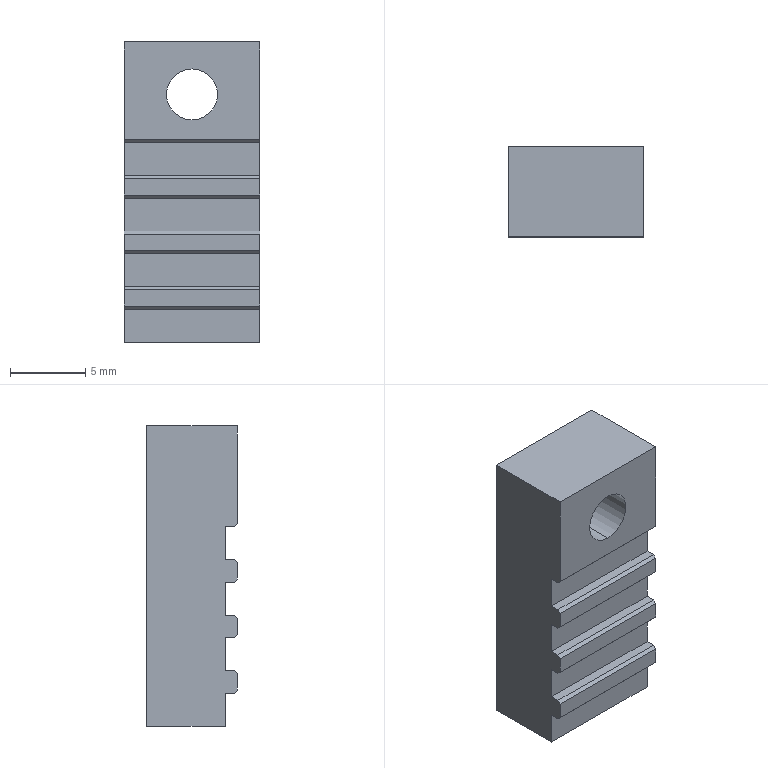Part | SolidWorks | mm | material A6061 | 1 solid | 32 faces | box 9 x 6 x 20 mm | volume 896 mm3 | plane 28 | cylinder 4 | commonest cylinder face diameters 6 x2 3.4 x2
Drawing notes:
0.20 X 45° CHAMFER TYP 7 PLCS - ALL GROOVE EDGES | from the solid: 7 inclined planes at 45° to y/z, size 9.0 x 0.2 x 0.2, at z=2.2, 3.5, 5.9, 7.2, 9.6, 10.9, 13.3
build123d program:
from build123d import *

# Parameters (mm, degrees)
SKETCH1_W                                       = 9
SKETCH1_H                                       = 20
BOSS_EXTRUDE1_DEPTH                             = 6
M3_HEX_SOCKET_HEAD_CAP_SCREW_CBORE1_D           = 3.4
M3_HEX_SOCKET_HEAD_CAP_SCREW_CBORE1_CBORE_D     = 6
M3_HEX_SOCKET_HEAD_CAP_SCREW_CBORE1_CBORE_DEPTH = 3.4
SKETCH5_W                                       = 2.2
SKETCH5_H                                       = 1.6
CUT_EXTRUDE1_DEPTH                              = 10
LPATTERN1_COUNT                                 = 4
LPATTERN1_PITCH                                 = 3.7
CHAMFER1_SIZE                                   = 0.2


with BuildPart() as part:
    # Sketch1 → Boss-Extrude1 (new body)
    with BuildSketch(Plane(origin=(0, 0, 0), x_dir=(1, 0, 0), z_dir=(0, 1, 0))):
        Rectangle(SKETCH1_W, SKETCH1_H)
    extrude(amount=BOSS_EXTRUDE1_DEPTH)

    # M3 Hex Socket Head Cap Screw CBORE1 (through all)
    with Locations(Plane(origin=(0, 6, 0), x_dir=(1, 0, 0), z_dir=(0, 1, 0))):
        with Locations((0, -6.5)):
            CounterBoreHole(M3_HEX_SOCKET_HEAD_CAP_SCREW_CBORE1_D / 2, M3_HEX_SOCKET_HEAD_CAP_SCREW_CBORE1_CBORE_D / 2, M3_HEX_SOCKET_HEAD_CAP_SCREW_CBORE1_CBORE_DEPTH)

    # Sketch5 → Cut-Extrude1 (cut)
    with BuildSketch(Plane(origin=(4.5, 0, 0), x_dir=(0, 0, -1), z_dir=(1, 0, 0))):
        with Locations((-2.2, 0)):
            Rectangle(SKETCH5_W, SKETCH5_H)
    cut_extrude1 = extrude(amount=-CUT_EXTRUDE1_DEPTH, mode=Mode.SUBTRACT)

    # LPattern1: Cut-Extrude1 ×4
    with Locations(*[(0, 0, -i * LPATTERN1_PITCH) for i in range(1, LPATTERN1_COUNT)]):
        add(cut_extrude1, mode=Mode.SUBTRACT)

    # Chamfer1
    chamfer1_edges = [part.edges().sort_by_distance(p)[0] for p in [
        (0, 0, 3.3),
        (0, 0, 1.1),
        (0, 0, -2.6),
        (0, 0, -0.4),
        (0, 0, -6.3),
        (0, 0, -4.1),
        (0, 0, -7.8),
    ]]
    chamfer(chamfer1_edges, length=CHAMFER1_SIZE)


solid = part.part
STEP:
#1=CARTESIAN_POINT('',(0.,2.6,3.5));
#2=VERTEX_POINT('',#1);
#3=CARTESIAN_POINT('',(0.,2.6,9.5));
#4=VERTEX_POINT('',#3);
#5=CARTESIAN_POINT('',(0.,2.6,6.5));
#6=DIRECTION('',(0.,1.,0.));
#7=DIRECTION('',(0.,0.,1.));
#8=AXIS2_PLACEMENT_3D('',#5,#6,#7);
#9=CIRCLE('',#8,3.);
#10=EDGE_CURVE('',#2,#4,#9,.T.);
#11=ORIENTED_EDGE('',*,*,#10,.F.);
#12=CARTESIAN_POINT('',(0.,6.,3.5));
#13=VERTEX_POINT('',#12);
#14=CARTESIAN_POINT('',(0.,6.,3.5));
#15=DIRECTION('',(0.,1.,0.));
#16=VECTOR('',#15,1000.);
#17=LINE('',#14,#16);
#18=EDGE_CURVE('',#2,#13,#17,.T.);
#19=ORIENTED_EDGE('',*,*,#18,.T.);
#20=CARTESIAN_POINT('',(0.,6.,9.5));
#21=VERTEX_POINT('',#20);
#22=CARTESIAN_POINT('',(0.,6.,6.5));
#23=DIRECTION('',(0.,1.,0.));
#24=DIRECTION('',(0.,0.,1.));
#25=AXIS2_PLACEMENT_3D('',#22,#23,#24);
#26=CIRCLE('',#25,3.);
#27=EDGE_CURVE('',#13,#21,#26,.T.);
#28=ORIENTED_EDGE('',*,*,#27,.T.);
#29=CARTESIAN_POINT('',(0.,6.,9.5));
#30=DIRECTION('',(0.,1.,0.));
#31=VECTOR('',#30,1000.);
#32=LINE('',#29,#31);
#33=EDGE_CURVE('',#4,#21,#32,.T.);
#34=ORIENTED_EDGE('',*,*,#33,.F.);
#35=EDGE_LOOP('',(#11,#19,#28,#34));
#36=FACE_OUTER_BOUND('',#35,.T.);
#37=CARTESIAN_POINT('',(0.,6.,6.5));
#38=DIRECTION('',(0.,1.,0.));
#39=DIRECTION('',(0.,0.,1.));
#40=AXIS2_PLACEMENT_3D('',#37,#38,#39);
#41=CYLINDRICAL_SURFACE('',#40,3.);
#42=ADVANCED_FACE('',(#36),#41,.F.);
#43=CARTESIAN_POINT('',(0.,0.,4.8));
#44=VERTEX_POINT('',#43);
#45=CARTESIAN_POINT('',(0.,0.,8.2));
#46=VERTEX_POINT('',#45);
#47=CARTESIAN_POINT('',(0.,0.,6.5));
#48=DIRECTION('',(0.,1.,0.));
#49=DIRECTION('',(0.,0.,1.));
#50=AXIS2_PLACEMENT_3D('',#47,#48,#49);
#51=CIRCLE('',#50,1.7);
#52=EDGE_CURVE('',#44,#46,#51,.T.);
#53=ORIENTED_EDGE('',*,*,#52,.F.);
#54=CARTESIAN_POINT('',(0.,2.6,4.8));
#55=VERTEX_POINT('',#54);
#56=CARTESIAN_POINT('',(0.,6.,4.8));
#57=DIRECTION('',(0.,1.,0.));
#58=VECTOR('',#57,1000.);
#59=LINE('',#56,#58);
#60=EDGE_CURVE('',#44,#55,#59,.T.);
#61=ORIENTED_EDGE('',*,*,#60,.T.);
#62=CARTESIAN_POINT('',(0.,2.6,8.2));
#63=VERTEX_POINT('',#62);
#64=CARTESIAN_POINT('',(0.,2.6,6.5));
#65=DIRECTION('',(0.,1.,0.));
#66=DIRECTION('',(0.,0.,1.));
#67=AXIS2_PLACEMENT_3D('',#64,#65,#66);
#68=CIRCLE('',#67,1.7);
#69=EDGE_CURVE('',#55,#63,#68,.T.);
#70=ORIENTED_EDGE('',*,*,#69,.T.);
#71=CARTESIAN_POINT('',(0.,6.,8.2));
#72=DIRECTION('',(0.,1.,0.));
#73=VECTOR('',#72,1000.);
#74=LINE('',#71,#73);
#75=EDGE_CURVE('',#46,#63,#74,.T.);
#76=ORIENTED_EDGE('',*,*,#75,.F.);
#77=EDGE_LOOP('',(#53,#61,#70,#76));
#78=FACE_OUTER_BOUND('',#77,.T.);
#79=CARTESIAN_POINT('',(0.,6.,6.5));
#80=DIRECTION('',(0.,1.,0.));
#81=DIRECTION('',(0.,0.,1.));
#82=AXIS2_PLACEMENT_3D('',#79,#80,#81);
#83=CYLINDRICAL_SURFACE('',#82,1.7);
#84=ADVANCED_FACE('',(#78),#83,.F.);
#85=CARTESIAN_POINT('',(-4.5,0.,-3.9));
#86=VERTEX_POINT('',#85);
#87=CARTESIAN_POINT('',(-4.5,0.,-2.8));
#88=VERTEX_POINT('',#87);
#89=CARTESIAN_POINT('',(-4.5,0.,10.));
#90=DIRECTION('',(0.,0.,1.));
#91=VECTOR('',#90,1000.);
#92=LINE('',#89,#91);
#93=EDGE_CURVE('',#86,#88,#92,.T.);
#94=ORIENTED_EDGE('',*,*,#93,.F.);
#95=CARTESIAN_POINT('',(4.5,0.,-3.9));
#96=VERTEX_POINT('',#95);
#97=CARTESIAN_POINT('',(4.5,0.,-3.9));
#98=DIRECTION('',(1.,0.,0.));
#99=VECTOR('',#98,1000.);
#100=LINE('',#97,#99);
#101=EDGE_CURVE('',#86,#96,#100,.T.);
#102=ORIENTED_EDGE('',*,*,#101,.T.);
#103=CARTESIAN_POINT('',(4.5,0.,-2.8));
#104=VERTEX_POINT('',#103);
#105=CARTESIAN_POINT('',(4.5,0.,10.));
#106=DIRECTION('',(0.,0.,-1.));
#107=VECTOR('',#106,1000.);
#108=LINE('',#105,#107);
#109=EDGE_CURVE('',#104,#96,#108,.T.);
#110=ORIENTED_EDGE('',*,*,#109,.F.);
#111=CARTESIAN_POINT('',(-4.5,0.,-2.8));
#112=DIRECTION('',(-1.,0.,0.));
#113=VECTOR('',#112,1000.);
#114=LINE('',#111,#113);
#115=EDGE_CURVE('',#104,#88,#114,.T.);
#116=ORIENTED_EDGE('',*,*,#115,.T.);
#117=EDGE_LOOP('',(#94,#102,#110,#116));
#118=FACE_OUTER_BOUND('',#117,.T.);
#119=CARTESIAN_POINT('',(0.,0.,0.));
#120=DIRECTION('',(0.,-1.,0.));
#121=DIRECTION('',(0.,0.,-1.));
#122=AXIS2_PLACEMENT_3D('',#119,#120,#121);
#123=PLANE('',#122);
#124=ADVANCED_FACE('',(#118),#123,.T.);
#125=CARTESIAN_POINT('',(-4.5,0.,-7.6));
#126=VERTEX_POINT('',#125);
#127=CARTESIAN_POINT('',(-4.5,0.,-6.5));
#128=VERTEX_POINT('',#127);
#129=CARTESIAN_POINT('',(-4.5,0.,10.));
#130=DIRECTION('',(0.,0.,1.));
#131=VECTOR('',#130,1000.);
#132=LINE('',#129,#131);
#133=EDGE_CURVE('',#126,#128,#132,.T.);
#134=ORIENTED_EDGE('',*,*,#133,.F.);
#135=CARTESIAN_POINT('',(4.5,0.,-7.6));
#136=VERTEX_POINT('',#135);
#137=CARTESIAN_POINT('',(4.5,0.,-7.6));
#138=DIRECTION('',(1.,0.,0.));
#139=VECTOR('',#138,1000.);
#140=LINE('',#137,#139);
#141=EDGE_CURVE('',#126,#136,#140,.T.);
#142=ORIENTED_EDGE('',*,*,#141,.T.);
#143=CARTESIAN_POINT('',(4.5,0.,-6.5));
#144=VERTEX_POINT('',#143);
#145=CARTESIAN_POINT('',(4.5,0.,10.));
#146=DIRECTION('',(0.,0.,-1.));
#147=VECTOR('',#146,1000.);
#148=LINE('',#145,#147);
#149=EDGE_CURVE('',#144,#136,#148,.T.);
#150=ORIENTED_EDGE('',*,*,#149,.F.);
#151=CARTESIAN_POINT('',(-4.5,0.,-6.5));
#152=DIRECTION('',(-1.,0.,0.));
#153=VECTOR('',#152,1000.);
#154=LINE('',#151,#153);
#155=EDGE_CURVE('',#144,#128,#154,.T.);
#156=ORIENTED_EDGE('',*,*,#155,.T.);
#157=EDGE_LOOP('',(#134,#142,#150,#156));
#158=FACE_OUTER_BOUND('',#157,.T.);
#159=CARTESIAN_POINT('',(0.,0.,0.));
#160=DIRECTION('',(0.,-1.,0.));
#161=DIRECTION('',(0.,0.,-1.));
#162=AXIS2_PLACEMENT_3D('',#159,#160,#161);
#163=PLANE('',#162);
#164=ADVANCED_FACE('',(#158),#163,.T.);
#165=CARTESIAN_POINT('',(-4.5,0.,-0.2));
#166=VERTEX_POINT('',#165);
#167=CARTESIAN_POINT('',(-4.5,0.,0.9));
#168=VERTEX_POINT('',#167);
#169=CARTESIAN_POINT('',(-4.5,0.,10.));
#170=DIRECTION('',(0.,0.,1.));
#171=VECTOR('',#170,1000.);
#172=LINE('',#169,#171);
#173=EDGE_CURVE('',#166,#168,#172,.T.);
#174=ORIENTED_EDGE('',*,*,#173,.F.);
#175=CARTESIAN_POINT('',(4.5,0.,-0.2));
#176=VERTEX_POINT('',#175);
#177=CARTESIAN_POINT('',(4.5,0.,-0.2));
#178=DIRECTION('',(1.,0.,0.));
#179=VECTOR('',#178,1000.);
#180=LINE('',#177,#179);
#181=EDGE_CURVE('',#166,#176,#180,.T.);
#182=ORIENTED_EDGE('',*,*,#181,.T.);
#183=CARTESIAN_POINT('',(4.5,0.,0.9));
#184=VERTEX_POINT('',#183);
#185=CARTESIAN_POINT('',(4.5,0.,10.));
#186=DIRECTION('',(0.,0.,-1.));
#187=VECTOR('',#186,1000.);
#188=LINE('',#185,#187);
#189=EDGE_CURVE('',#184,#176,#188,.T.);
#190=ORIENTED_EDGE('',*,*,#189,.F.);
#191=CARTESIAN_POINT('',(-4.5,0.,0.9));
#192=DIRECTION('',(-1.,0.,0.));
#193=VECTOR('',#192,1000.);
#194=LINE('',#191,#193);
#195=EDGE_CURVE('',#184,#168,#194,.T.);
#196=ORIENTED_EDGE('',*,*,#195,.T.);
#197=EDGE_LOOP('',(#174,#182,#190,#196));
#198=FACE_OUTER_BOUND('',#197,.T.);
#199=CARTESIAN_POINT('',(0.,0.,0.));
#200=DIRECTION('',(0.,-1.,0.));
#201=DIRECTION('',(0.,0.,-1.));
#202=AXIS2_PLACEMENT_3D('',#199,#200,#201);
#203=PLANE('',#202);
#204=ADVANCED_FACE('',(#198),#203,.T.);
#205=ORIENTED_EDGE('',*,*,#149,.T.);
#206=CARTESIAN_POINT('',(4.5,0.2,-7.8));
#207=VERTEX_POINT('',#206);
#208=CARTESIAN_POINT('',(4.5,0.2,-7.8));
#209=DIRECTION('',(0.,0.7071,-0.7071));
#210=VECTOR('',#209,1000.);
#211=LINE('',#208,#210);
#212=EDGE_CURVE('',#136,#207,#211,.T.);
#213=ORIENTED_EDGE('',*,*,#212,.T.);
#214=CARTESIAN_POINT('',(4.5,0.8,-7.8));
#215=VERTEX_POINT('',#214);
#216=CARTESIAN_POINT('',(4.5,-0.8,-7.8));
#217=DIRECTION('',(0.,-1.,0.));
#218=VECTOR('',#217,1000.);
#219=LINE('',#216,#218);
#220=EDGE_CURVE('',#215,#207,#219,.T.);
#221=ORIENTED_EDGE('',*,*,#220,.F.);
#222=CARTESIAN_POINT('',(4.5,0.8,-10.));
#223=VERTEX_POINT('',#222);
#224=CARTESIAN_POINT('',(4.5,0.8,-7.8));
#225=DIRECTION('',(0.,0.,1.));
#226=VECTOR('',#225,1000.);
#227=LINE('',#224,#226);
#228=EDGE_CURVE('',#223,#215,#227,.T.);
#229=ORIENTED_EDGE('',*,*,#228,.F.);
#230=CARTESIAN_POINT('',(4.5,6.,-10.));
#231=VERTEX_POINT('',#230);
#232=CARTESIAN_POINT('',(4.5,6.,-10.));
#233=DIRECTION('',(0.,-1.,0.));
#234=VECTOR('',#233,1000.);
#235=LINE('',#232,#234);
#236=EDGE_CURVE('',#231,#223,#235,.T.);
#237=ORIENTED_EDGE('',*,*,#236,.F.);
#238=CARTESIAN_POINT('',(4.5,6.,10.));
#239=VERTEX_POINT('',#238);
#240=CARTESIAN_POINT('',(4.5,6.,10.));
#241=DIRECTION('',(0.,0.,-1.));
#242=VECTOR('',#241,1000.);
#243=LINE('',#240,#242);
#244=EDGE_CURVE('',#239,#231,#243,.T.);
#245=ORIENTED_EDGE('',*,*,#244,.F.);
#246=CARTESIAN_POINT('',(4.5,0.,10.));
#247=VERTEX_POINT('',#246);
#248=CARTESIAN_POINT('',(4.5,6.,10.));
#249=DIRECTION('',(0.,-1.,0.));
#250=VECTOR('',#249,1000.);
#251=LINE('',#248,#250);
#252=EDGE_CURVE('',#239,#247,#251,.T.);
#253=ORIENTED_EDGE('',*,*,#252,.T.);
#254=CARTESIAN_POINT('',(4.5,0.,3.5));
#255=VERTEX_POINT('',#254);
#256=CARTESIAN_POINT('',(4.5,0.,10.));
#257=DIRECTION('',(0.,0.,-1.));
#258=VECTOR('',#257,1000.);
#259=LINE('',#256,#258);
#260=EDGE_CURVE('',#247,#255,#259,.T.);
#261=ORIENTED_EDGE('',*,*,#260,.T.);
#262=CARTESIAN_POINT('',(4.5,0.2,3.3));
#263=VERTEX_POINT('',#262);
#264=CARTESIAN_POINT('',(4.5,0.2,3.3));
#265=DIRECTION('',(0.,0.7071,-0.7071));
#266=VECTOR('',#265,1000.);
#267=LINE('',#264,#266);
#268=EDGE_CURVE('',#255,#263,#267,.T.);
#269=ORIENTED_EDGE('',*,*,#268,.T.);
#270=CARTESIAN_POINT('',(4.5,0.8,3.3));
#271=VERTEX_POINT('',#270);
#272=CARTESIAN_POINT('',(4.5,-0.8,3.3));
#273=DIRECTION('',(0.,-1.,0.));
#274=VECTOR('',#273,1000.);
#275=LINE('',#272,#274);
#276=EDGE_CURVE('',#271,#263,#275,.T.);
#277=ORIENTED_EDGE('',*,*,#276,.F.);
#278=CARTESIAN_POINT('',(4.5,0.8,1.1));
#279=VERTEX_POINT('',#278);
#280=CARTESIAN_POINT('',(4.5,0.8,3.3));
#281=DIRECTION('',(0.,0.,1.));
#282=VECTOR('',#281,1000.);
#283=LINE('',#280,#282);
#284=EDGE_CURVE('',#279,#271,#283,.T.);
#285=ORIENTED_EDGE('',*,*,#284,.F.);
#286=CARTESIAN_POINT('',(4.5,0.2,1.1));
#287=VERTEX_POINT('',#286);
#288=CARTESIAN_POINT('',(4.5,-0.8,1.1));
#289=DIRECTION('',(0.,1.,0.));
#290=VECTOR('',#289,1000.);
#291=LINE('',#288,#290);
#292=EDGE_CURVE('',#287,#279,#291,.T.);
#293=ORIENTED_EDGE('',*,*,#292,.F.);
#294=CARTESIAN_POINT('',(4.5,0.2,1.1));
#295=DIRECTION('',(0.,-0.7071,-0.7071));
#296=VECTOR('',#295,1000.);
#297=LINE('',#294,#296);
#298=EDGE_CURVE('',#287,#184,#297,.T.);
#299=ORIENTED_EDGE('',*,*,#298,.T.);
#300=ORIENTED_EDGE('',*,*,#189,.T.);
#301=CARTESIAN_POINT('',(4.5,0.2,-0.4));
#302=VERTEX_POINT('',#301);
#303=CARTESIAN_POINT('',(4.5,0.2,-0.4));
#304=DIRECTION('',(0.,0.7071,-0.7071));
#305=VECTOR('',#304,1000.);
#306=LINE('',#303,#305);
#307=EDGE_CURVE('',#176,#302,#306,.T.);
#308=ORIENTED_EDGE('',*,*,#307,.T.);
#309=CARTESIAN_POINT('',(4.5,0.8,-0.4));
#310=VERTEX_POINT('',#309);
#311=CARTESIAN_POINT('',(4.5,-0.8,-0.4));
#312=DIRECTION('',(0.,-1.,0.));
#313=VECTOR('',#312,1000.);
#314=LINE('',#311,#313);
#315=EDGE_CURVE('',#310,#302,#314,.T.);
#316=ORIENTED_EDGE('',*,*,#315,.F.);
#317=CARTESIAN_POINT('',(4.5,0.8,-2.6));
#318=VERTEX_POINT('',#317);
#319=CARTESIAN_POINT('',(4.5,0.8,-0.4));
#320=DIRECTION('',(0.,0.,1.));
#321=VECTOR('',#320,1000.);
#322=LINE('',#319,#321);
#323=EDGE_CURVE('',#318,#310,#322,.T.);
#324=ORIENTED_EDGE('',*,*,#323,.F.);
#325=CARTESIAN_POINT('',(4.5,0.2,-2.6));
#326=VERTEX_POINT('',#325);
#327=CARTESIAN_POINT('',(4.5,-0.8,-2.6));
#328=DIRECTION('',(0.,1.,0.));
#329=VECTOR('',#328,1000.);
#330=LINE('',#327,#329);
#331=EDGE_CURVE('',#326,#318,#330,.T.);
#332=ORIENTED_EDGE('',*,*,#331,.F.);
#333=CARTESIAN_POINT('',(4.5,0.2,-2.6));
#334=DIRECTION('',(0.,-0.7071,-0.7071));
#335=VECTOR('',#334,1000.);
#336=LINE('',#333,#335);
#337=EDGE_CURVE('',#326,#104,#336,.T.);
#338=ORIENTED_EDGE('',*,*,#337,.T.);
#339=ORIENTED_EDGE('',*,*,#109,.T.);
#340=CARTESIAN_POINT('',(4.5,0.2,-4.1));
#341=VERTEX_POINT('',#340);
#342=CARTESIAN_POINT('',(4.5,0.2,-4.1));
#343=DIRECTION('',(0.,0.7071,-0.7071));
#344=VECTOR('',#343,1000.);
#345=LINE('',#342,#344);
#346=EDGE_CURVE('',#96,#341,#345,.T.);
#347=ORIENTED_EDGE('',*,*,#346,.T.);
#348=CARTESIAN_POINT('',(4.5,0.8,-4.1));
#349=VERTEX_POINT('',#348);
#350=CARTESIAN_POINT('',(4.5,-0.8,-4.1));
#351=DIRECTION('',(0.,-1.,0.));
#352=VECTOR('',#351,1000.);
#353=LINE('',#350,#352);
#354=EDGE_CURVE('',#349,#341,#353,.T.);
#355=ORIENTED_EDGE('',*,*,#354,.F.);
#356=CARTESIAN_POINT('',(4.5,0.8,-6.3));
#357=VERTEX_POINT('',#356);
#358=CARTESIAN_POINT('',(4.5,0.8,-4.1));
#359=DIRECTION('',(0.,0.,1.));
#360=VECTOR('',#359,1000.);
#361=LINE('',#358,#360);
#362=EDGE_CURVE('',#357,#349,#361,.T.);
#363=ORIENTED_EDGE('',*,*,#362,.F.);
#364=CARTESIAN_POINT('',(4.5,0.2,-6.3));
#365=VERTEX_POINT('',#364);
#366=CARTESIAN_POINT('',(4.5,-0.8,-6.3));
#367=DIRECTION('',(0.,1.,0.));
#368=VECTOR('',#367,1000.);
#369=LINE('',#366,#368);
#370=EDGE_CURVE('',#365,#357,#369,.T.);
#371=ORIENTED_EDGE('',*,*,#370,.F.);
#372=CARTESIAN_POINT('',(4.5,0.2,-6.3));
#373=DIRECTION('',(0.,-0.7071,-0.7071));
#374=VECTOR('',#373,1000.);
#375=LINE('',#372,#374);
#376=EDGE_CURVE('',#365,#144,#375,.T.);
#377=ORIENTED_EDGE('',*,*,#376,.T.);
#378=EDGE_LOOP('',(#205,#213,#221,#229,#237,#245,#253,#261,#269,#277,#285,#293,#299,#300,#308,#316,#324,#332,#338,#339,#347,#355,#363,#371,#377));
#379=FACE_OUTER_BOUND('',#378,.T.);
#380=CARTESIAN_POINT('',(4.5,6.,10.));
#381=DIRECTION('',(-1.,0.,0.));
#382=DIRECTION('',(0.,0.,1.));
#383=AXIS2_PLACEMENT_3D('',#380,#381,#382);
#384=PLANE('',#383);
#385=ADVANCED_FACE('',(#379),#384,.F.);
#386=ORIENTED_EDGE('',*,*,#236,.T.);
#387=CARTESIAN_POINT('',(-4.5,0.8,-10.));
#388=VERTEX_POINT('',#387);
#389=CARTESIAN_POINT('',(-5.5,0.8,-10.));
#390=DIRECTION('',(1.,0.,0.));
#391=VECTOR('',#390,1000.);
#392=LINE('',#389,#391);
#393=EDGE_CURVE('',#388,#223,#392,.T.);
#394=ORIENTED_EDGE('',*,*,#393,.F.);
#395=CARTESIAN_POINT('',(-4.5,6.,-10.));
#396=VERTEX_POINT('',#395);
#397=CARTESIAN_POINT('',(-4.5,6.,-10.));
#398=DIRECTION('',(0.,-1.,0.));
#399=VECTOR('',#398,1000.);
#400=LINE('',#397,#399);
#401=EDGE_CURVE('',#396,#388,#400,.T.);
#402=ORIENTED_EDGE('',*,*,#401,.F.);
#403=CARTESIAN_POINT('',(-4.5,6.,-10.));
#404=DIRECTION('',(-1.,0.,0.));
#405=VECTOR('',#404,1000.);
#406=LINE('',#403,#405);
#407=EDGE_CURVE('',#231,#396,#406,.T.);
#408=ORIENTED_EDGE('',*,*,#407,.F.);
#409=EDGE_LOOP('',(#386,#394,#402,#408));
#410=FACE_OUTER_BOUND('',#409,.T.);
#411=CARTESIAN_POINT('',(-4.5,6.,-10.));
#412=DIRECTION('',(0.,0.,1.));
#413=DIRECTION('',(1.,0.,0.));
#414=AXIS2_PLACEMENT_3D('',#411,#412,#413);
#415=PLANE('',#414);
#416=ADVANCED_FACE('',(#410),#415,.F.);
#417=CARTESIAN_POINT('',(-4.5,0.8,-7.8));
#418=VERTEX_POINT('',#417);
#419=CARTESIAN_POINT('',(-4.5,0.2,-7.8));
#420=VERTEX_POINT('',#419);
#421=CARTESIAN_POINT('',(-4.5,6.,-7.8));
#422=DIRECTION('',(0.,-1.,0.));
#423=VECTOR('',#422,1000.);
#424=LINE('',#421,#423);
#425=EDGE_CURVE('',#418,#420,#424,.T.);
#426=ORIENTED_EDGE('',*,*,#425,.T.);
#427=CARTESIAN_POINT('',(-4.5,0.2,-7.8));
#428=DIRECTION('',(0.,-0.7071,0.7071));
#429=VECTOR('',#428,1000.);
#430=LINE('',#427,#429);
#431=EDGE_CURVE('',#420,#126,#430,.T.);
#432=ORIENTED_EDGE('',*,*,#431,.T.);
#433=ORIENTED_EDGE('',*,*,#133,.T.);
#434=CARTESIAN_POINT('',(-4.5,0.2,-6.3));
#435=VERTEX_POINT('',#434);
#436=CARTESIAN_POINT('',(-4.5,0.2,-6.3));
#437=DIRECTION('',(0.,0.7071,0.7071));
#438=VECTOR('',#437,1000.);
#439=LINE('',#436,#438);
#440=EDGE_CURVE('',#128,#435,#439,.T.);
#441=ORIENTED_EDGE('',*,*,#440,.T.);
#442=CARTESIAN_POINT('',(-4.5,0.8,-6.3));
#443=VERTEX_POINT('',#442);
#444=CARTESIAN_POINT('',(-4.5,6.,-6.3));
#445=DIRECTION('',(0.,1.,0.));
#446=VECTOR('',#445,1000.);
#447=LINE('',#444,#446);
#448=EDGE_CURVE('',#435,#443,#447,.T.);
#449=ORIENTED_EDGE('',*,*,#448,.T.);
#450=CARTESIAN_POINT('',(-4.5,0.8,-4.1));
#451=VERTEX_POINT('',#450);
#452=CARTESIAN_POINT('',(-4.5,0.8,10.));
#453=DIRECTION('',(0.,0.,1.));
#454=VECTOR('',#453,1000.);
#455=LINE('',#452,#454);
#456=EDGE_CURVE('',#443,#451,#455,.T.);
#457=ORIENTED_EDGE('',*,*,#456,.T.);
#458=CARTESIAN_POINT('',(-4.5,0.2,-4.1));
#459=VERTEX_POINT('',#458);
#460=CARTESIAN_POINT('',(-4.5,6.,-4.1));
#461=DIRECTION('',(0.,-1.,0.));
#462=VECTOR('',#461,1000.);
#463=LINE('',#460,#462);
#464=EDGE_CURVE('',#451,#459,#463,.T.);
#465=ORIENTED_EDGE('',*,*,#464,.T.);
#466=CARTESIAN_POINT('',(-4.5,0.2,-4.1));
#467=DIRECTION('',(0.,-0.7071,0.7071));
#468=VECTOR('',#467,1000.);
#469=LINE('',#466,#468);
#470=EDGE_CURVE('',#459,#86,#469,.T.);
#471=ORIENTED_EDGE('',*,*,#470,.T.);
#472=ORIENTED_EDGE('',*,*,#93,.T.);
#473=CARTESIAN_POINT('',(-4.5,0.2,-2.6));
#474=VERTEX_POINT('',#473);
#475=CARTESIAN_POINT('',(-4.5,0.2,-2.6));
#476=DIRECTION('',(0.,0.7071,0.7071));
#477=VECTOR('',#476,1000.);
#478=LINE('',#475,#477);
#479=EDGE_CURVE('',#88,#474,#478,.T.);
#480=ORIENTED_EDGE('',*,*,#479,.T.);
#481=CARTESIAN_POINT('',(-4.5,0.8,-2.6));
#482=VERTEX_POINT('',#481);
#483=CARTESIAN_POINT('',(-4.5,6.,-2.6));
#484=DIRECTION('',(0.,1.,0.));
#485=VECTOR('',#484,1000.);
#486=LINE('',#483,#485);
#487=EDGE_CURVE('',#474,#482,#486,.T.);
#488=ORIENTED_EDGE('',*,*,#487,.T.);
#489=CARTESIAN_POINT('',(-4.5,0.8,-0.4));
#490=VERTEX_POINT('',#489);
#491=CARTESIAN_POINT('',(-4.5,0.8,10.));
#492=DIRECTION('',(0.,0.,1.));
#493=VECTOR('',#492,1000.);
#494=LINE('',#491,#493);
#495=EDGE_CURVE('',#482,#490,#494,.T.);
#496=ORIENTED_EDGE('',*,*,#495,.T.);
#497=CARTESIAN_POINT('',(-4.5,0.2,-0.4));
#498=VERTEX_POINT('',#497);
#499=CARTESIAN_POINT('',(-4.5,6.,-0.4));
#500=DIRECTION('',(0.,-1.,0.));
#501=VECTOR('',#500,1000.);
#502=LINE('',#499,#501);
#503=EDGE_CURVE('',#490,#498,#502,.T.);
#504=ORIENTED_EDGE('',*,*,#503,.T.);
#505=CARTESIAN_POINT('',(-4.5,0.2,-0.4));
#506=DIRECTION('',(0.,-0.7071,0.7071));
#507=VECTOR('',#506,1000.);
#508=LINE('',#505,#507);
#509=EDGE_CURVE('',#498,#166,#508,.T.);
#510=ORIENTED_EDGE('',*,*,#509,.T.);
#511=ORIENTED_EDGE('',*,*,#173,.T.);
#512=CARTESIAN_POINT('',(-4.5,0.2,1.1));
#513=VERTEX_POINT('',#512);
#514=CARTESIAN_POINT('',(-4.5,0.2,1.1));
#515=DIRECTION('',(0.,0.7071,0.7071));
#516=VECTOR('',#515,1000.);
#517=LINE('',#514,#516);
#518=EDGE_CURVE('',#168,#513,#517,.T.);
#519=ORIENTED_EDGE('',*,*,#518,.T.);
#520=CARTESIAN_POINT('',(-4.5,0.8,1.1));
#521=VERTEX_POINT('',#520);
#522=CARTESIAN_POINT('',(-4.5,6.,1.1));
#523=DIRECTION('',(0.,1.,0.));
#524=VECTOR('',#523,1000.);
#525=LINE('',#522,#524);
#526=EDGE_CURVE('',#513,#521,#525,.T.);
#527=ORIENTED_EDGE('',*,*,#526,.T.);
#528=CARTESIAN_POINT('',(-4.5,0.8,3.3));
#529=VERTEX_POINT('',#528);
#530=CARTESIAN_POINT('',(-4.5,0.8,10.));
#531=DIRECTION('',(0.,0.,1.));
#532=VECTOR('',#531,1000.);
#533=LINE('',#530,#532);
#534=EDGE_CURVE('',#521,#529,#533,.T.);
#535=ORIENTED_EDGE('',*,*,#534,.T.);
#536=CARTESIAN_POINT('',(-4.5,0.2,3.3));
#537=VERTEX_POINT('',#536);
#538=CARTESIAN_POINT('',(-4.5,6.,3.3));
#539=DIRECTION('',(0.,-1.,0.));
#540=VECTOR('',#539,1000.);
#541=LINE('',#538,#540);
#542=EDGE_CURVE('',#529,#537,#541,.T.);
#543=ORIENTED_EDGE('',*,*,#542,.T.);
#544=CARTESIAN_POINT('',(-4.5,0.,3.5));
#545=VERTEX_POINT('',#544);
#546=CARTESIAN_POINT('',(-4.5,0.2,3.3));
#547=DIRECTION('',(0.,-0.7071,0.7071));
#548=VECTOR('',#547,1000.);
#549=LINE('',#546,#548);
#550=EDGE_CURVE('',#537,#545,#549,.T.);
#551=ORIENTED_EDGE('',*,*,#550,.T.);
#552=CARTESIAN_POINT('',(-4.5,0.,10.));
#553=VERTEX_POINT('',#552);
#554=CARTESIAN_POINT('',(-4.5,0.,10.));
#555=DIRECTION('',(0.,0.,1.));
#556=VECTOR('',#555,1000.);
#557=LINE('',#554,#556);
#558=EDGE_CURVE('',#545,#553,#557,.T.);
#559=ORIENTED_EDGE('',*,*,#558,.T.);
#560=CARTESIAN_POINT('',(-4.5,6.,10.));
#561=VERTEX_POINT('',#560);
#562=CARTESIAN_POINT('',(-4.5,6.,10.));
#563=DIRECTION('',(0.,-1.,0.));
#564=VECTOR('',#563,1000.);
#565=LINE('',#562,#564);
#566=EDGE_CURVE('',#561,#553,#565,.T.);
#567=ORIENTED_EDGE('',*,*,#566,.F.);
#568=CARTESIAN_POINT('',(-4.5,6.,10.));
#569=DIRECTION('',(0.,0.,1.));
#570=VECTOR('',#569,1000.);
#571=LINE('',#568,#570);
#572=EDGE_CURVE('',#396,#561,#571,.T.);
#573=ORIENTED_EDGE('',*,*,#572,.F.);
#574=ORIENTED_EDGE('',*,*,#401,.T.);
#575=CARTESIAN_POINT('',(-4.5,0.8,10.));
#576=DIRECTION('',(0.,0.,1.));
#577=VECTOR('',#576,1000.);
#578=LINE('',#575,#577);
#579=EDGE_CURVE('',#388,#418,#578,.T.);
#580=ORIENTED_EDGE('',*,*,#579,.T.);
#581=EDGE_LOOP('',(#426,#432,#433,#441,#449,#457,#465,#471,#472,#480,#488,#496,#504,#510,#511,#519,#527,#535,#543,#551,#559,#567,#573,#574,#580));
#582=FACE_OUTER_BOUND('',#581,.T.);
#583=CARTESIAN_POINT('',(-4.5,6.,10.));
#584=DIRECTION('',(1.,0.,0.));
#585=DIRECTION('',(0.,0.,-1.));
#586=AXIS2_PLACEMENT_3D('',#583,#584,#585);
#587=PLANE('',#586);
#588=ADVANCED_FACE('',(#582),#587,.F.);
#589=CARTESIAN_POINT('',(-4.5,0.,10.));
#590=DIRECTION('',(1.,0.,0.));
#591=VECTOR('',#590,1000.);
#592=LINE('',#589,#591);
#593=EDGE_CURVE('',#553,#247,#592,.T.);
#594=ORIENTED_EDGE('',*,*,#593,.T.);
#595=ORIENTED_EDGE('',*,*,#252,.F.);
#596=CARTESIAN_POINT('',(-4.5,6.,10.));
#597=DIRECTION('',(1.,0.,0.));
#598=VECTOR('',#597,1000.);
#599=LINE('',#596,#598);
#600=EDGE_CURVE('',#561,#239,#599,.T.);
#601=ORIENTED_EDGE('',*,*,#600,.F.);
#602=ORIENTED_EDGE('',*,*,#566,.T.);
#603=EDGE_LOOP('',(#594,#595,#601,#602));
#604=FACE_OUTER_BOUND('',#603,.T.);
#605=CARTESIAN_POINT('',(-4.5,6.,10.));
#606=DIRECTION('',(0.,0.,-1.));
#607=DIRECTION('',(-1.,0.,0.));
#608=AXIS2_PLACEMENT_3D('',#605,#606,#607);
#609=PLANE('',#608);
#610=ADVANCED_FACE('',(#604),#609,.F.);
#611=CARTESIAN_POINT('',(0.,6.,6.5));
#612=DIRECTION('',(0.,1.,0.));
#613=DIRECTION('',(0.,0.,1.));
#614=AXIS2_PLACEMENT_3D('',#611,#612,#613);
#615=CIRCLE('',#614,3.);
#616=EDGE_CURVE('',#21,#13,#615,.T.);
#617=ORIENTED_EDGE('',*,*,#616,.F.);
#618=ORIENTED_EDGE('',*,*,#27,.F.);
#619=EDGE_LOOP('',(#617,#618));
#620=FACE_BOUND('',#619,.T.);
#621=ORIENTED_EDGE('',*,*,#244,.T.);
#622=ORIENTED_EDGE('',*,*,#407,.T.);
#623=ORIENTED_EDGE('',*,*,#572,.T.);
#624=ORIENTED_EDGE('',*,*,#600,.T.);
#625=EDGE_LOOP('',(#621,#622,#623,#624));
#626=FACE_OUTER_BOUND('',#625,.T.);
#627=CARTESIAN_POINT('',(0.,6.,0.));
#628=DIRECTION('',(0.,-1.,0.));
#629=DIRECTION('',(0.,0.,-1.));
#630=AXIS2_PLACEMENT_3D('',#627,#628,#629);
#631=PLANE('',#630);
#632=ADVANCED_FACE('',(#620,#626),#631,.F.);
#633=ORIENTED_EDGE('',*,*,#558,.F.);
#634=CARTESIAN_POINT('',(4.5,0.,3.5));
#635=DIRECTION('',(1.,0.,0.));
#636=VECTOR('',#635,1000.);
#637=LINE('',#634,#636);
#638=EDGE_CURVE('',#545,#255,#637,.T.);
#639=ORIENTED_EDGE('',*,*,#638,.T.);
#640=ORIENTED_EDGE('',*,*,#260,.F.);
#641=ORIENTED_EDGE('',*,*,#593,.F.);
#642=EDGE_LOOP('',(#633,#639,#640,#641));
#643=FACE_OUTER_BOUND('',#642,.T.);
#644=CARTESIAN_POINT('',(0.,0.,6.5));
#645=DIRECTION('',(0.,1.,0.));
#646=DIRECTION('',(0.,0.,1.));
#647=AXIS2_PLACEMENT_3D('',#644,#645,#646);
#648=CIRCLE('',#647,1.7);
#649=EDGE_CURVE('',#46,#44,#648,.T.);
#650=ORIENTED_EDGE('',*,*,#649,.T.);
#651=ORIENTED_EDGE('',*,*,#52,.T.);
#652=EDGE_LOOP('',(#650,#651));
#653=FACE_BOUND('',#652,.T.);
#654=CARTESIAN_POINT('',(0.,0.,0.));
#655=DIRECTION('',(0.,-1.,0.));
#656=DIRECTION('',(0.,0.,-1.));
#657=AXIS2_PLACEMENT_3D('',#654,#655,#656);
#658=PLANE('',#657);
#659=ADVANCED_FACE('',(#643,#653),#658,.T.);
#660=ORIENTED_EDGE('',*,*,#60,.F.);
#661=ORIENTED_EDGE('',*,*,#649,.F.);
#662=ORIENTED_EDGE('',*,*,#75,.T.);
#663=CARTESIAN_POINT('',(0.,2.6,6.5));
#664=DIRECTION('',(0.,1.,0.));
#665=DIRECTION('',(0.,0.,1.));
#666=AXIS2_PLACEMENT_3D('',#663,#664,#665);
#667=CIRCLE('',#666,1.7);
#668=EDGE_CURVE('',#63,#55,#667,.T.);
#669=ORIENTED_EDGE('',*,*,#668,.T.);
#670=EDGE_LOOP('',(#660,#661,#662,#669));
#671=FACE_OUTER_BOUND('',#670,.T.);
#672=CARTESIAN_POINT('',(0.,6.,6.5));
#673=DIRECTION('',(0.,1.,0.));
#674=DIRECTION('',(0.,0.,1.));
#675=AXIS2_PLACEMENT_3D('',#672,#673,#674);
#676=CYLINDRICAL_SURFACE('',#675,1.7);
#677=ADVANCED_FACE('',(#671),#676,.F.);
#678=ORIENTED_EDGE('',*,*,#668,.F.);
#679=ORIENTED_EDGE('',*,*,#69,.F.);
#680=EDGE_LOOP('',(#678,#679));
#681=FACE_BOUND('',#680,.T.);
#682=CARTESIAN_POINT('',(0.,2.6,6.5));
#683=DIRECTION('',(0.,1.,0.));
#684=DIRECTION('',(0.,0.,1.));
#685=AXIS2_PLACEMENT_3D('',#682,#683,#684);
#686=CIRCLE('',#685,3.);
#687=EDGE_CURVE('',#4,#2,#686,.T.);
#688=ORIENTED_EDGE('',*,*,#687,.T.);
#689=ORIENTED_EDGE('',*,*,#10,.T.);
#690=EDGE_LOOP('',(#688,#689));
#691=FACE_OUTER_BOUND('',#690,.T.);
#692=CARTESIAN_POINT('',(1.7,2.6,6.5));
#693=DIRECTION('',(0.,-1.,0.));
#694=DIRECTION('',(0.,0.,-1.));
#695=AXIS2_PLACEMENT_3D('',#692,#693,#694);
#696=PLANE('',#695);
#697=ADVANCED_FACE('',(#681,#691),#696,.F.);
#698=ORIENTED_EDGE('',*,*,#18,.F.);
#699=ORIENTED_EDGE('',*,*,#687,.F.);
#700=ORIENTED_EDGE('',*,*,#33,.T.);
#701=ORIENTED_EDGE('',*,*,#616,.T.);
#702=EDGE_LOOP('',(#698,#699,#700,#701));
#703=FACE_OUTER_BOUND('',#702,.T.);
#704=CARTESIAN_POINT('',(0.,6.,6.5));
#705=DIRECTION('',(0.,1.,0.));
#706=DIRECTION('',(0.,0.,1.));
#707=AXIS2_PLACEMENT_3D('',#704,#705,#706);
#708=CYLINDRICAL_SURFACE('',#707,3.);
#709=ADVANCED_FACE('',(#703),#708,.F.);
#710=CARTESIAN_POINT('',(-5.5,0.8,1.1));
#711=DIRECTION('',(1.,0.,0.));
#712=VECTOR('',#711,1000.);
#713=LINE('',#710,#712);
#714=EDGE_CURVE('',#521,#279,#713,.T.);
#715=ORIENTED_EDGE('',*,*,#714,.T.);
#716=ORIENTED_EDGE('',*,*,#284,.T.);
#717=CARTESIAN_POINT('',(-5.5,0.8,3.3));
#718=DIRECTION('',(1.,0.,0.));
#719=VECTOR('',#718,1000.);
#720=LINE('',#717,#719);
#721=EDGE_CURVE('',#529,#271,#720,.T.);
#722=ORIENTED_EDGE('',*,*,#721,.F.);
#723=ORIENTED_EDGE('',*,*,#534,.F.);
#724=EDGE_LOOP('',(#715,#716,#722,#723));
#725=FACE_OUTER_BOUND('',#724,.T.);
#726=CARTESIAN_POINT('',(-5.5,0.8,3.3));
#727=DIRECTION('',(0.,1.,0.));
#728=DIRECTION('',(0.,0.,1.));
#729=AXIS2_PLACEMENT_3D('',#726,#727,#728);
#730=PLANE('',#729);
#731=ADVANCED_FACE('',(#725),#730,.F.);
#732=ORIENTED_EDGE('',*,*,#526,.F.);
#733=CARTESIAN_POINT('',(4.5,0.2,1.1));
#734=DIRECTION('',(1.,0.,0.));
#735=VECTOR('',#734,1000.);
#736=LINE('',#733,#735);
#737=EDGE_CURVE('',#513,#287,#736,.T.);
#738=ORIENTED_EDGE('',*,*,#737,.T.);
#739=ORIENTED_EDGE('',*,*,#292,.T.);
#740=ORIENTED_EDGE('',*,*,#714,.F.);
#741=EDGE_LOOP('',(#732,#738,#739,#740));
#742=FACE_OUTER_BOUND('',#741,.T.);
#743=CARTESIAN_POINT('',(-5.5,-0.8,1.1));
#744=DIRECTION('',(0.,0.,-1.));
#745=DIRECTION('',(-1.,0.,0.));
#746=AXIS2_PLACEMENT_3D('',#743,#744,#745);
#747=PLANE('',#746);
#748=ADVANCED_FACE('',(#742),#747,.F.);
#749=ORIENTED_EDGE('',*,*,#276,.T.);
#750=CARTESIAN_POINT('',(-4.5,0.2,3.3));
#751=DIRECTION('',(-1.,0.,0.));
#752=VECTOR('',#751,1000.);
#753=LINE('',#750,#752);
#754=EDGE_CURVE('',#263,#537,#753,.T.);
#755=ORIENTED_EDGE('',*,*,#754,.T.);
#756=ORIENTED_EDGE('',*,*,#542,.F.);
#757=ORIENTED_EDGE('',*,*,#721,.T.);
#758=EDGE_LOOP('',(#749,#755,#756,#757));
#759=FACE_OUTER_BOUND('',#758,.T.);
#760=CARTESIAN_POINT('',(-5.5,-0.8,3.3));
#761=DIRECTION('',(0.,0.,1.));
#762=DIRECTION('',(1.,0.,0.));
#763=AXIS2_PLACEMENT_3D('',#760,#761,#762);
#764=PLANE('',#763);
#765=ADVANCED_FACE('',(#759),#764,.F.);
#766=ORIENTED_EDGE('',*,*,#393,.T.);
#767=ORIENTED_EDGE('',*,*,#228,.T.);
#768=CARTESIAN_POINT('',(-5.5,0.8,-7.8));
#769=DIRECTION('',(1.,0.,0.));
#770=VECTOR('',#769,1000.);
#771=LINE('',#768,#770);
#772=EDGE_CURVE('',#418,#215,#771,.T.);
#773=ORIENTED_EDGE('',*,*,#772,.F.);
#774=ORIENTED_EDGE('',*,*,#579,.F.);
#775=EDGE_LOOP('',(#766,#767,#773,#774));
#776=FACE_OUTER_BOUND('',#775,.T.);
#777=CARTESIAN_POINT('',(-5.5,0.8,-7.8));
#778=DIRECTION('',(0.,1.,0.));
#779=DIRECTION('',(0.,0.,1.));
#780=AXIS2_PLACEMENT_3D('',#777,#778,#779);
#781=PLANE('',#780);
#782=ADVANCED_FACE('',(#776),#781,.F.);
#783=ORIENTED_EDGE('',*,*,#220,.T.);
#784=CARTESIAN_POINT('',(-4.5,0.2,-7.8));
#785=DIRECTION('',(-1.,0.,0.));
#786=VECTOR('',#785,1000.);
#787=LINE('',#784,#786);
#788=EDGE_CURVE('',#207,#420,#787,.T.);
#789=ORIENTED_EDGE('',*,*,#788,.T.);
#790=ORIENTED_EDGE('',*,*,#425,.F.);
#791=ORIENTED_EDGE('',*,*,#772,.T.);
#792=EDGE_LOOP('',(#783,#789,#790,#791));
#793=FACE_OUTER_BOUND('',#792,.T.);
#794=CARTESIAN_POINT('',(-5.5,-0.8,-7.8));
#795=DIRECTION('',(0.,0.,1.));
#796=DIRECTION('',(1.,0.,0.));
#797=AXIS2_PLACEMENT_3D('',#794,#795,#796);
#798=PLANE('',#797);
#799=ADVANCED_FACE('',(#793),#798,.F.);
#800=CARTESIAN_POINT('',(-5.5,0.8,-6.3));
#801=DIRECTION('',(1.,0.,0.));
#802=VECTOR('',#801,1000.);
#803=LINE('',#800,#802);
#804=EDGE_CURVE('',#443,#357,#803,.T.);
#805=ORIENTED_EDGE('',*,*,#804,.T.);
#806=ORIENTED_EDGE('',*,*,#362,.T.);
#807=CARTESIAN_POINT('',(-5.5,0.8,-4.1));
#808=DIRECTION('',(1.,0.,0.));
#809=VECTOR('',#808,1000.);
#810=LINE('',#807,#809);
#811=EDGE_CURVE('',#451,#349,#810,.T.);
#812=ORIENTED_EDGE('',*,*,#811,.F.);
#813=ORIENTED_EDGE('',*,*,#456,.F.);
#814=EDGE_LOOP('',(#805,#806,#812,#813));
#815=FACE_OUTER_BOUND('',#814,.T.);
#816=CARTESIAN_POINT('',(-5.5,0.8,-4.1));
#817=DIRECTION('',(0.,1.,0.));
#818=DIRECTION('',(0.,0.,1.));
#819=AXIS2_PLACEMENT_3D('',#816,#817,#818);
#820=PLANE('',#819);
#821=ADVANCED_FACE('',(#815),#820,.F.);
#822=ORIENTED_EDGE('',*,*,#448,.F.);
#823=CARTESIAN_POINT('',(4.5,0.2,-6.3));
#824=DIRECTION('',(1.,0.,0.));
#825=VECTOR('',#824,1000.);
#826=LINE('',#823,#825);
#827=EDGE_CURVE('',#435,#365,#826,.T.);
#828=ORIENTED_EDGE('',*,*,#827,.T.);
#829=ORIENTED_EDGE('',*,*,#370,.T.);
#830=ORIENTED_EDGE('',*,*,#804,.F.);
#831=EDGE_LOOP('',(#822,#828,#829,#830));
#832=FACE_OUTER_BOUND('',#831,.T.);
#833=CARTESIAN_POINT('',(-5.5,-0.8,-6.3));
#834=DIRECTION('',(0.,0.,-1.));
#835=DIRECTION('',(-1.,0.,0.));
#836=AXIS2_PLACEMENT_3D('',#833,#834,#835);
#837=PLANE('',#836);
#838=ADVANCED_FACE('',(#832),#837,.F.);
#839=ORIENTED_EDGE('',*,*,#354,.T.);
#840=CARTESIAN_POINT('',(-4.5,0.2,-4.1));
#841=DIRECTION('',(-1.,0.,0.));
#842=VECTOR('',#841,1000.);
#843=LINE('',#840,#842);
#844=EDGE_CURVE('',#341,#459,#843,.T.);
#845=ORIENTED_EDGE('',*,*,#844,.T.);
#846=ORIENTED_EDGE('',*,*,#464,.F.);
#847=ORIENTED_EDGE('',*,*,#811,.T.);
#848=EDGE_LOOP('',(#839,#845,#846,#847));
#849=FACE_OUTER_BOUND('',#848,.T.);
#850=CARTESIAN_POINT('',(-5.5,-0.8,-4.1));
#851=DIRECTION('',(0.,0.,1.));
#852=DIRECTION('',(1.,0.,0.));
#853=AXIS2_PLACEMENT_3D('',#850,#851,#852);
#854=PLANE('',#853);
#855=ADVANCED_FACE('',(#849),#854,.F.);
#856=CARTESIAN_POINT('',(-5.5,0.8,-2.6));
#857=DIRECTION('',(1.,0.,0.));
#858=VECTOR('',#857,1000.);
#859=LINE('',#856,#858);
#860=EDGE_CURVE('',#482,#318,#859,.T.);
#861=ORIENTED_EDGE('',*,*,#860,.T.);
#862=ORIENTED_EDGE('',*,*,#323,.T.);
#863=CARTESIAN_POINT('',(-5.5,0.8,-0.4));
#864=DIRECTION('',(1.,0.,0.));
#865=VECTOR('',#864,1000.);
#866=LINE('',#863,#865);
#867=EDGE_CURVE('',#490,#310,#866,.T.);
#868=ORIENTED_EDGE('',*,*,#867,.F.);
#869=ORIENTED_EDGE('',*,*,#495,.F.);
#870=EDGE_LOOP('',(#861,#862,#868,#869));
#871=FACE_OUTER_BOUND('',#870,.T.);
#872=CARTESIAN_POINT('',(-5.5,0.8,-0.4));
#873=DIRECTION('',(0.,1.,0.));
#874=DIRECTION('',(0.,0.,1.));
#875=AXIS2_PLACEMENT_3D('',#872,#873,#874);
#876=PLANE('',#875);
#877=ADVANCED_FACE('',(#871),#876,.F.);
#878=ORIENTED_EDGE('',*,*,#487,.F.);
#879=CARTESIAN_POINT('',(4.5,0.2,-2.6));
#880=DIRECTION('',(1.,0.,0.));
#881=VECTOR('',#880,1000.);
#882=LINE('',#879,#881);
#883=EDGE_CURVE('',#474,#326,#882,.T.);
#884=ORIENTED_EDGE('',*,*,#883,.T.);
#885=ORIENTED_EDGE('',*,*,#331,.T.);
#886=ORIENTED_EDGE('',*,*,#860,.F.);
#887=EDGE_LOOP('',(#878,#884,#885,#886));
#888=FACE_OUTER_BOUND('',#887,.T.);
#889=CARTESIAN_POINT('',(-5.5,-0.8,-2.6));
#890=DIRECTION('',(0.,0.,-1.));
#891=DIRECTION('',(-1.,0.,0.));
#892=AXIS2_PLACEMENT_3D('',#889,#890,#891);
#893=PLANE('',#892);
#894=ADVANCED_FACE('',(#888),#893,.F.);
#895=ORIENTED_EDGE('',*,*,#315,.T.);
#896=CARTESIAN_POINT('',(-4.5,0.2,-0.4));
#897=DIRECTION('',(-1.,0.,0.));
#898=VECTOR('',#897,1000.);
#899=LINE('',#896,#898);
#900=EDGE_CURVE('',#302,#498,#899,.T.);
#901=ORIENTED_EDGE('',*,*,#900,.T.);
#902=ORIENTED_EDGE('',*,*,#503,.F.);
#903=ORIENTED_EDGE('',*,*,#867,.T.);
#904=EDGE_LOOP('',(#895,#901,#902,#903));
#905=FACE_OUTER_BOUND('',#904,.T.);
#906=CARTESIAN_POINT('',(-5.5,-0.8,-0.4));
#907=DIRECTION('',(0.,0.,1.));
#908=DIRECTION('',(1.,0.,0.));
#909=AXIS2_PLACEMENT_3D('',#906,#907,#908);
#910=PLANE('',#909);
#911=ADVANCED_FACE('',(#905),#910,.F.);
#912=ORIENTED_EDGE('',*,*,#212,.F.);
#913=ORIENTED_EDGE('',*,*,#141,.F.);
#914=ORIENTED_EDGE('',*,*,#431,.F.);
#915=ORIENTED_EDGE('',*,*,#788,.F.);
#916=EDGE_LOOP('',(#912,#913,#914,#915));
#917=FACE_OUTER_BOUND('',#916,.T.);
#918=CARTESIAN_POINT('',(-5.5,0.2,-7.8));
#919=DIRECTION('',(0.,-0.7071,-0.7071));
#920=DIRECTION('',(1.,0.,0.));
#921=AXIS2_PLACEMENT_3D('',#918,#919,#920);
#922=PLANE('',#921);
#923=ADVANCED_FACE('',(#917),#922,.T.);
#924=ORIENTED_EDGE('',*,*,#440,.F.);
#925=ORIENTED_EDGE('',*,*,#155,.F.);
#926=ORIENTED_EDGE('',*,*,#376,.F.);
#927=ORIENTED_EDGE('',*,*,#827,.F.);
#928=EDGE_LOOP('',(#924,#925,#926,#927));
#929=FACE_OUTER_BOUND('',#928,.T.);
#930=CARTESIAN_POINT('',(-5.5,0.2,-6.3));
#931=DIRECTION('',(0.,-0.7071,0.7071));
#932=DIRECTION('',(-1.,0.,0.));
#933=AXIS2_PLACEMENT_3D('',#930,#931,#932);
#934=PLANE('',#933);
#935=ADVANCED_FACE('',(#929),#934,.T.);
#936=ORIENTED_EDGE('',*,*,#346,.F.);
#937=ORIENTED_EDGE('',*,*,#101,.F.);
#938=ORIENTED_EDGE('',*,*,#470,.F.);
#939=ORIENTED_EDGE('',*,*,#844,.F.);
#940=EDGE_LOOP('',(#936,#937,#938,#939));
#941=FACE_OUTER_BOUND('',#940,.T.);
#942=CARTESIAN_POINT('',(-5.5,0.2,-4.1));
#943=DIRECTION('',(0.,-0.7071,-0.7071));
#944=DIRECTION('',(1.,0.,0.));
#945=AXIS2_PLACEMENT_3D('',#942,#943,#944);
#946=PLANE('',#945);
#947=ADVANCED_FACE('',(#941),#946,.T.);
#948=ORIENTED_EDGE('',*,*,#479,.F.);
#949=ORIENTED_EDGE('',*,*,#115,.F.);
#950=ORIENTED_EDGE('',*,*,#337,.F.);
#951=ORIENTED_EDGE('',*,*,#883,.F.);
#952=EDGE_LOOP('',(#948,#949,#950,#951));
#953=FACE_OUTER_BOUND('',#952,.T.);
#954=CARTESIAN_POINT('',(-5.5,0.2,-2.6));
#955=DIRECTION('',(0.,-0.7071,0.7071));
#956=DIRECTION('',(-1.,0.,0.));
#957=AXIS2_PLACEMENT_3D('',#954,#955,#956);
#958=PLANE('',#957);
#959=ADVANCED_FACE('',(#953),#958,.T.);
#960=ORIENTED_EDGE('',*,*,#307,.F.);
#961=ORIENTED_EDGE('',*,*,#181,.F.);
#962=ORIENTED_EDGE('',*,*,#509,.F.);
#963=ORIENTED_EDGE('',*,*,#900,.F.);
#964=EDGE_LOOP('',(#960,#961,#962,#963));
#965=FACE_OUTER_BOUND('',#964,.T.);
#966=CARTESIAN_POINT('',(-5.5,0.2,-0.4));
#967=DIRECTION('',(0.,-0.7071,-0.7071));
#968=DIRECTION('',(1.,0.,0.));
#969=AXIS2_PLACEMENT_3D('',#966,#967,#968);
#970=PLANE('',#969);
#971=ADVANCED_FACE('',(#965),#970,.T.);
#972=ORIENTED_EDGE('',*,*,#518,.F.);
#973=ORIENTED_EDGE('',*,*,#195,.F.);
#974=ORIENTED_EDGE('',*,*,#298,.F.);
#975=ORIENTED_EDGE('',*,*,#737,.F.);
#976=EDGE_LOOP('',(#972,#973,#974,#975));
#977=FACE_OUTER_BOUND('',#976,.T.);
#978=CARTESIAN_POINT('',(-5.5,0.2,1.1));
#979=DIRECTION('',(0.,-0.7071,0.7071));
#980=DIRECTION('',(-1.,0.,0.));
#981=AXIS2_PLACEMENT_3D('',#978,#979,#980);
#982=PLANE('',#981);
#983=ADVANCED_FACE('',(#977),#982,.T.);
#984=ORIENTED_EDGE('',*,*,#268,.F.);
#985=ORIENTED_EDGE('',*,*,#638,.F.);
#986=ORIENTED_EDGE('',*,*,#550,.F.);
#987=ORIENTED_EDGE('',*,*,#754,.F.);
#988=EDGE_LOOP('',(#984,#985,#986,#987));
#989=FACE_OUTER_BOUND('',#988,.T.);
#990=CARTESIAN_POINT('',(-5.5,0.2,3.3));
#991=DIRECTION('',(0.,-0.7071,-0.7071));
#992=DIRECTION('',(1.,0.,0.));
#993=AXIS2_PLACEMENT_3D('',#990,#991,#992);
#994=PLANE('',#993);
#995=ADVANCED_FACE('',(#989),#994,.T.);
#996=CLOSED_SHELL('',(#42,#84,#124,#164,#204,#385,#416,#588,#610,#632,#659,#677,#697,#709,#731,#748,#765,#782,#799,#821,#838,#855,#877,#894,#911,#923,#935,#947,#959,#971,#983,#995));
#997=MANIFOLD_SOLID_BREP('',#996);
#998=CARTESIAN_POINT('',(0.,0.,0.));
#999=DIRECTION('',(0.,0.,1.));
#1000=DIRECTION('',(1.,0.,0.));
#1001=AXIS2_PLACEMENT_3D('',#998,#999,#1000);
#1002=(LENGTH_UNIT()NAMED_UNIT(*)SI_UNIT(.MILLI.,.METRE.));
#1003=UNCERTAINTY_MEASURE_WITH_UNIT(LENGTH_MEASURE(0.00001),#1002,'','');
#1004=(NAMED_UNIT(*)PLANE_ANGLE_UNIT()SI_UNIT($,.RADIAN.));
#1005=(NAMED_UNIT(*)SI_UNIT($,.STERADIAN.)SOLID_ANGLE_UNIT());
#1006=(GEOMETRIC_REPRESENTATION_CONTEXT(3)GLOBAL_UNCERTAINTY_ASSIGNED_CONTEXT((#1003))GLOBAL_UNIT_ASSIGNED_CONTEXT((#1002,#1004,#1005))REPRESENTATION_CONTEXT('',''));
#1007=ADVANCED_BREP_SHAPE_REPRESENTATION('',(#997,#1001),#1006);